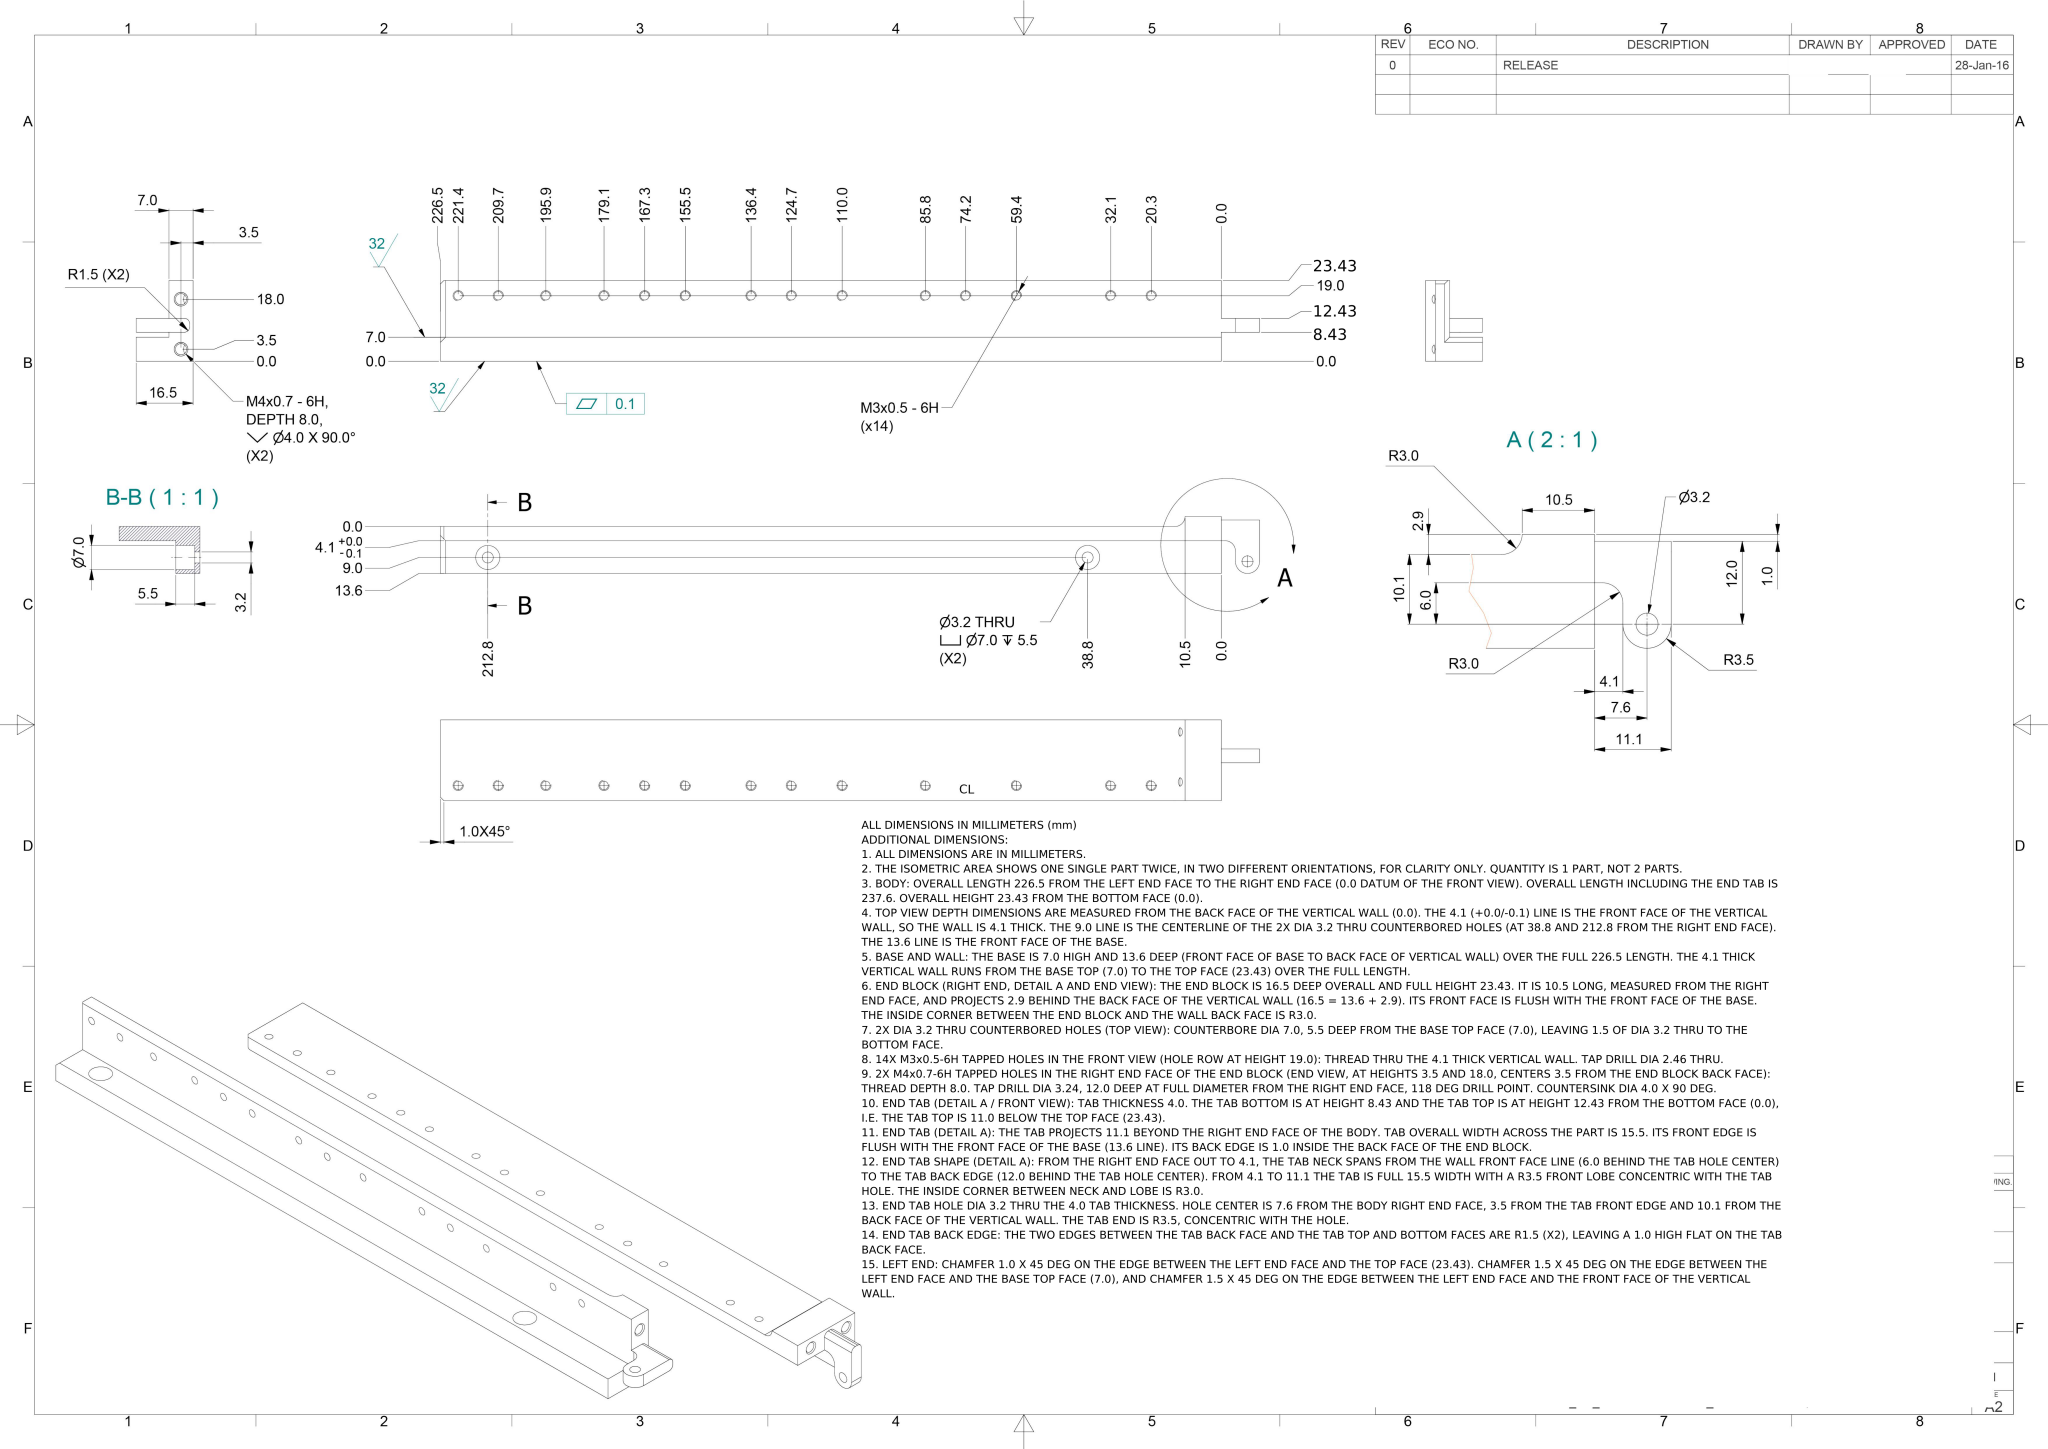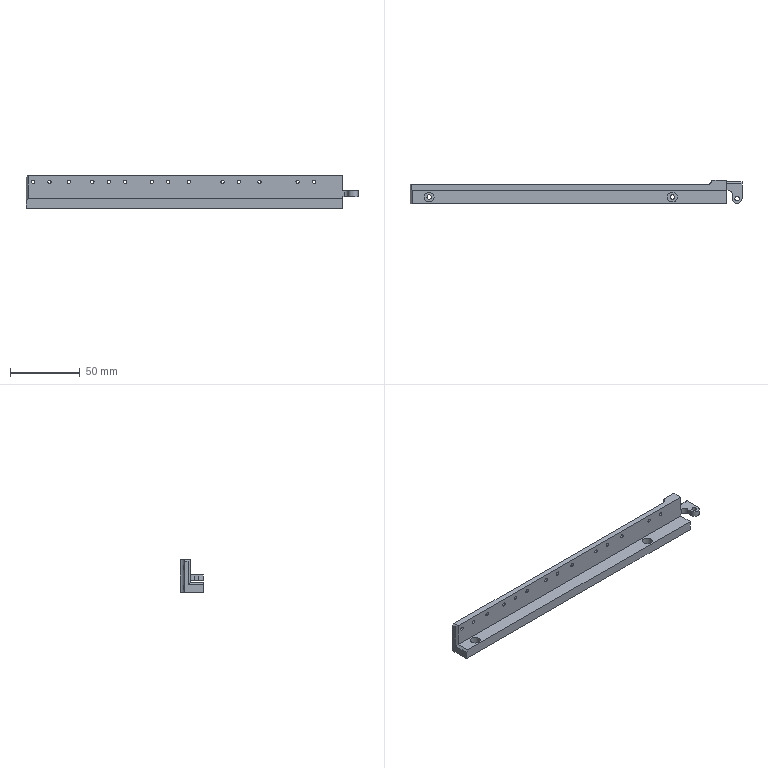Part | NX | mm | 1 solid | 49 faces | box 237.6 x 16.5 x 23.43 mm | volume 37103 mm3 | cylinder 26 | plane 19 | cone 4 | commonest cylinder face diameters 2.459 x14 7 x3 3.2 x3 3.242 x2 6 x2 3 x2